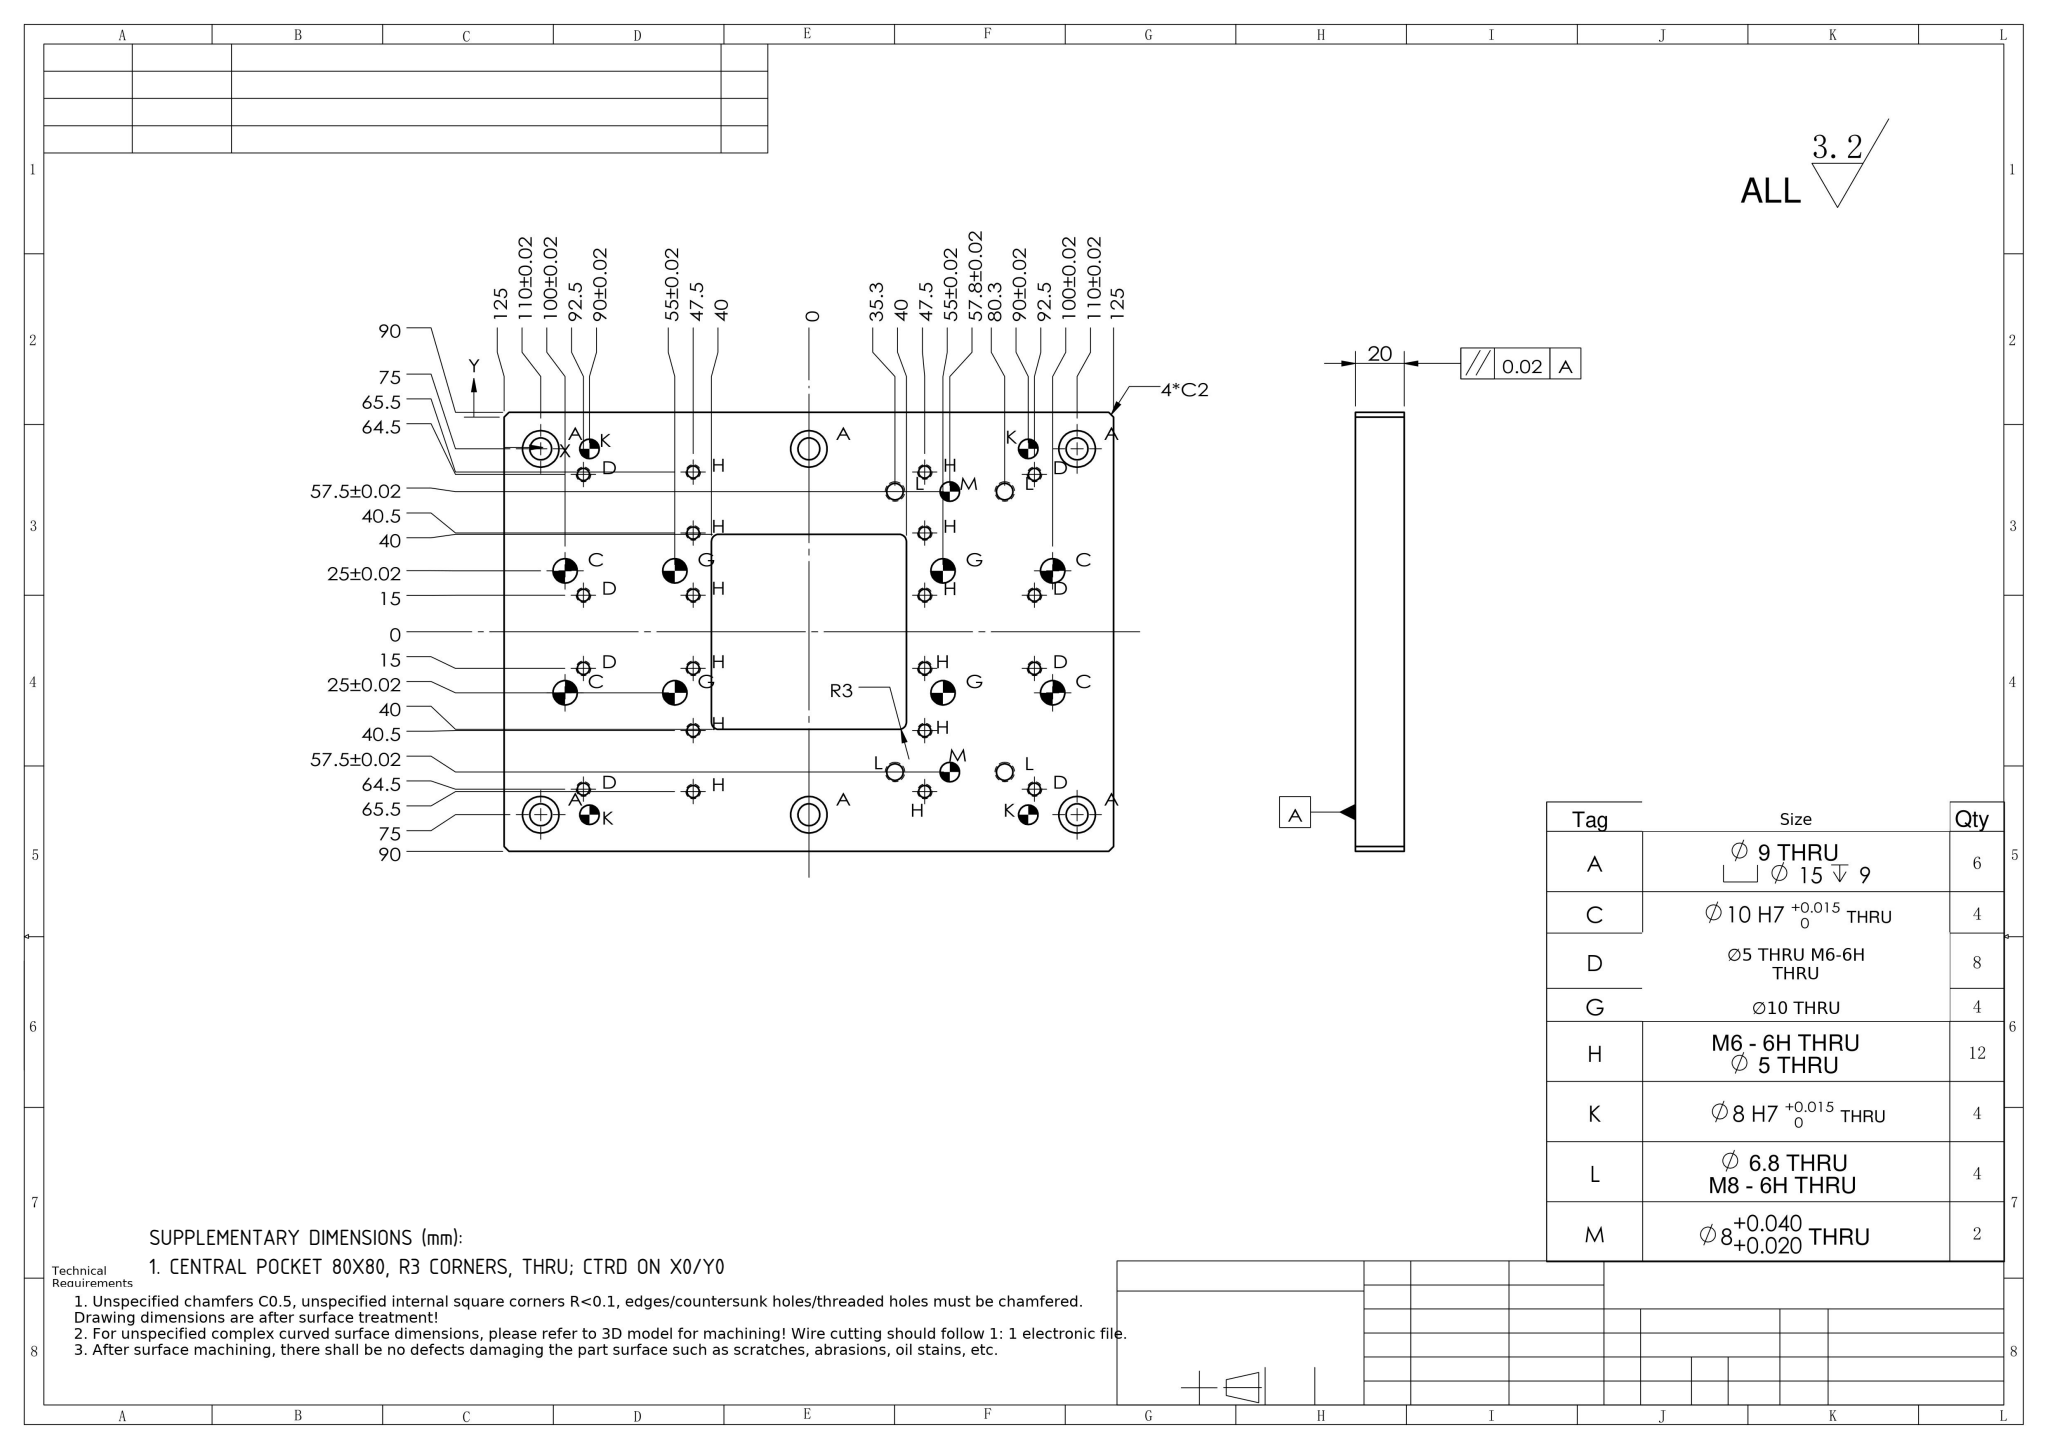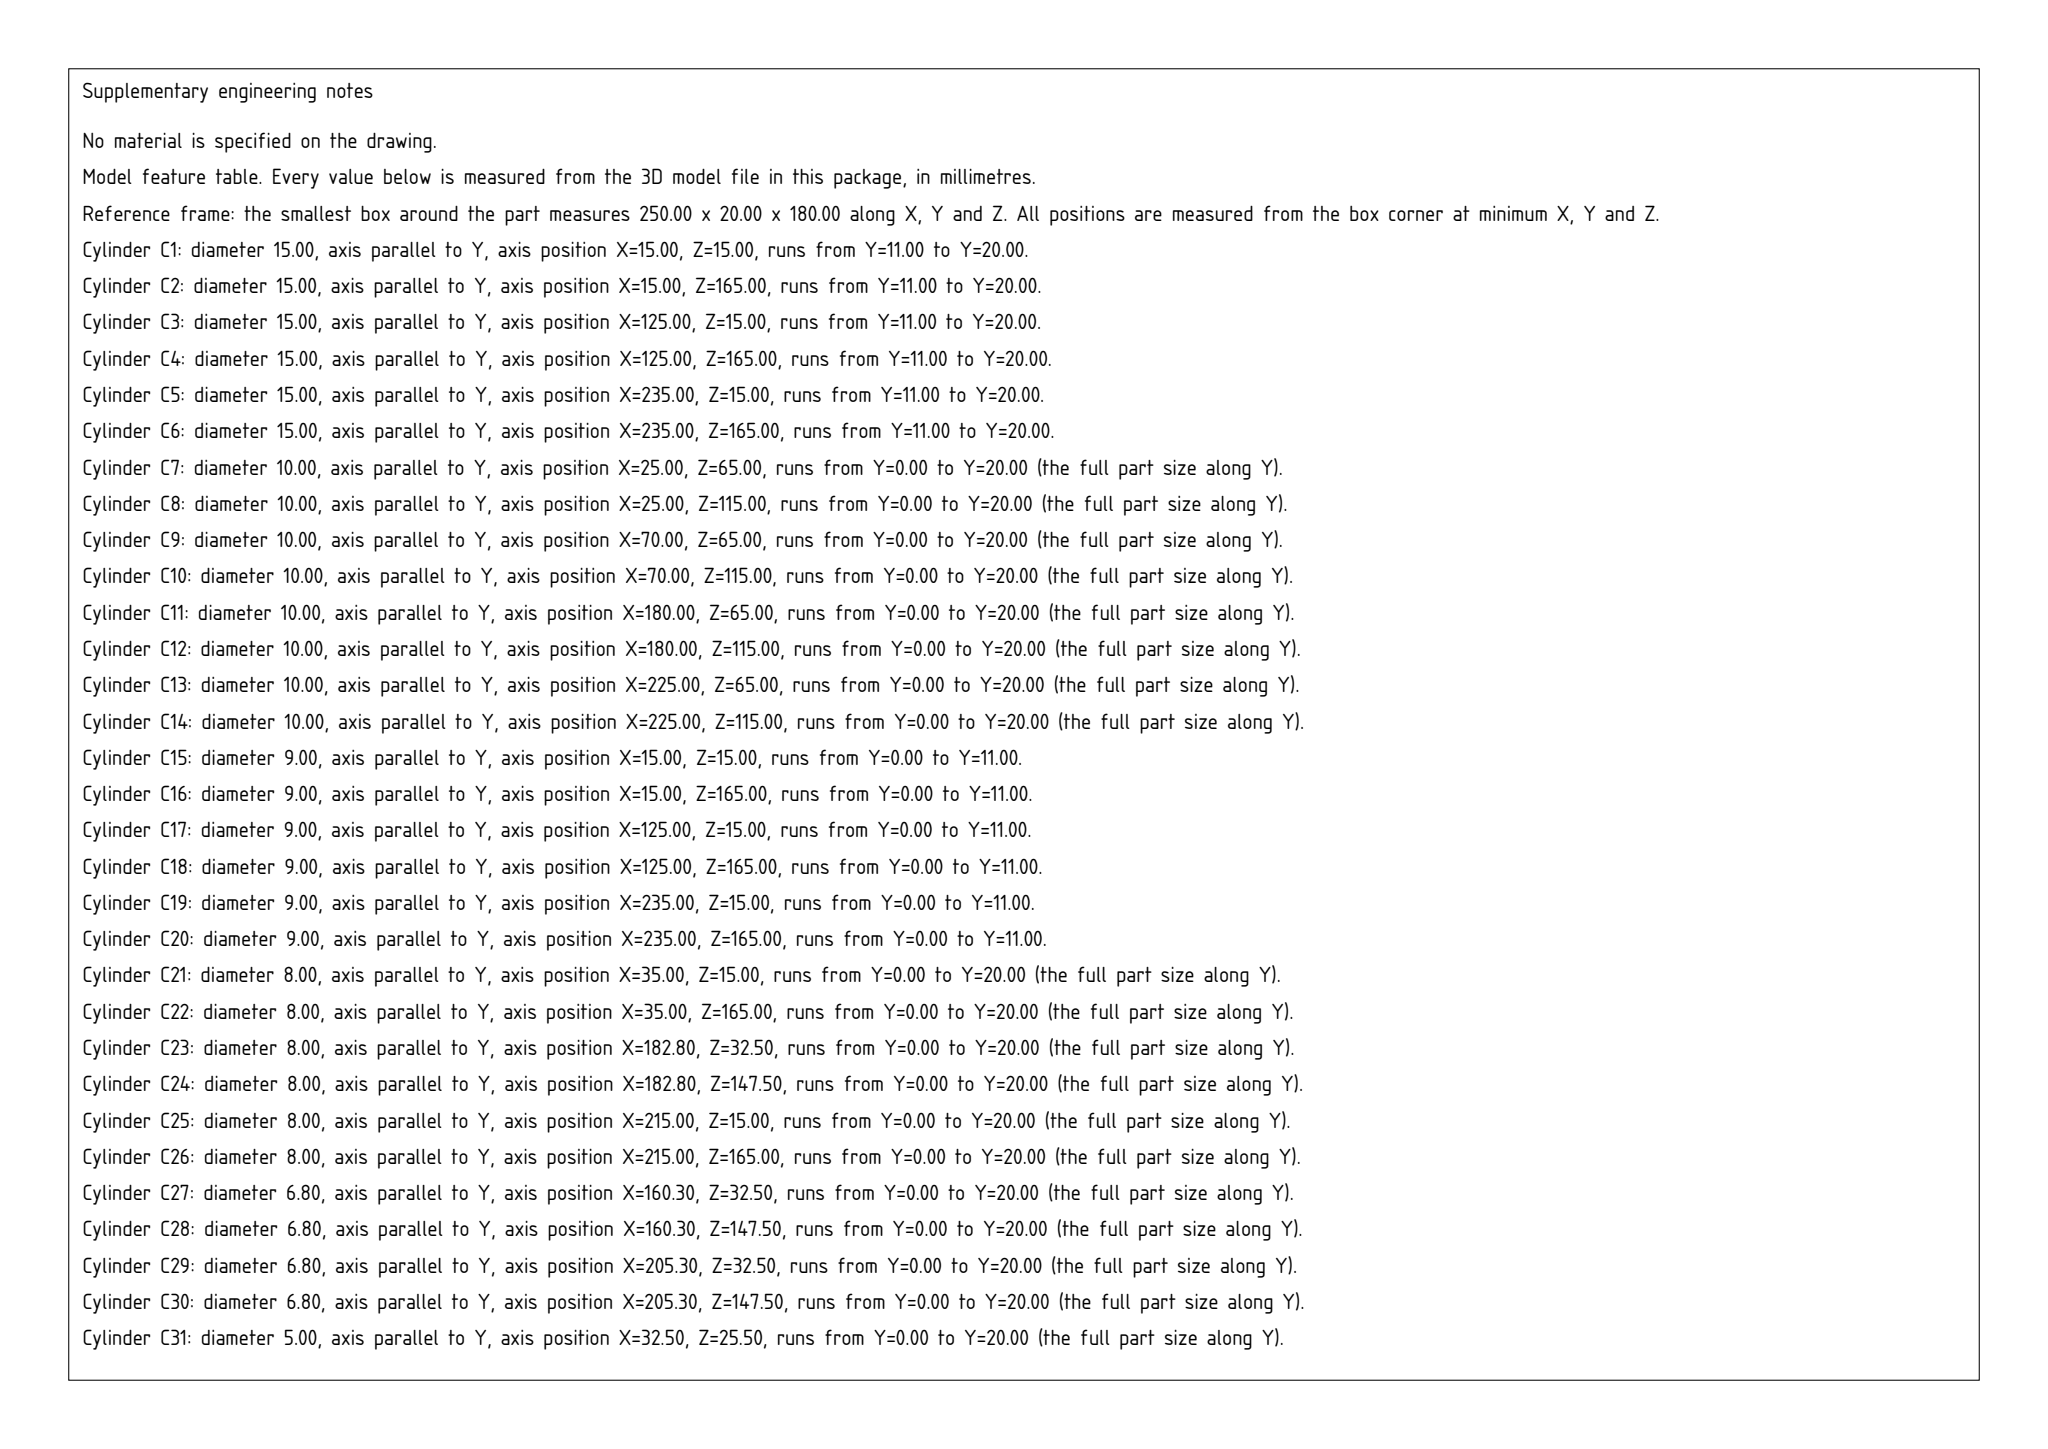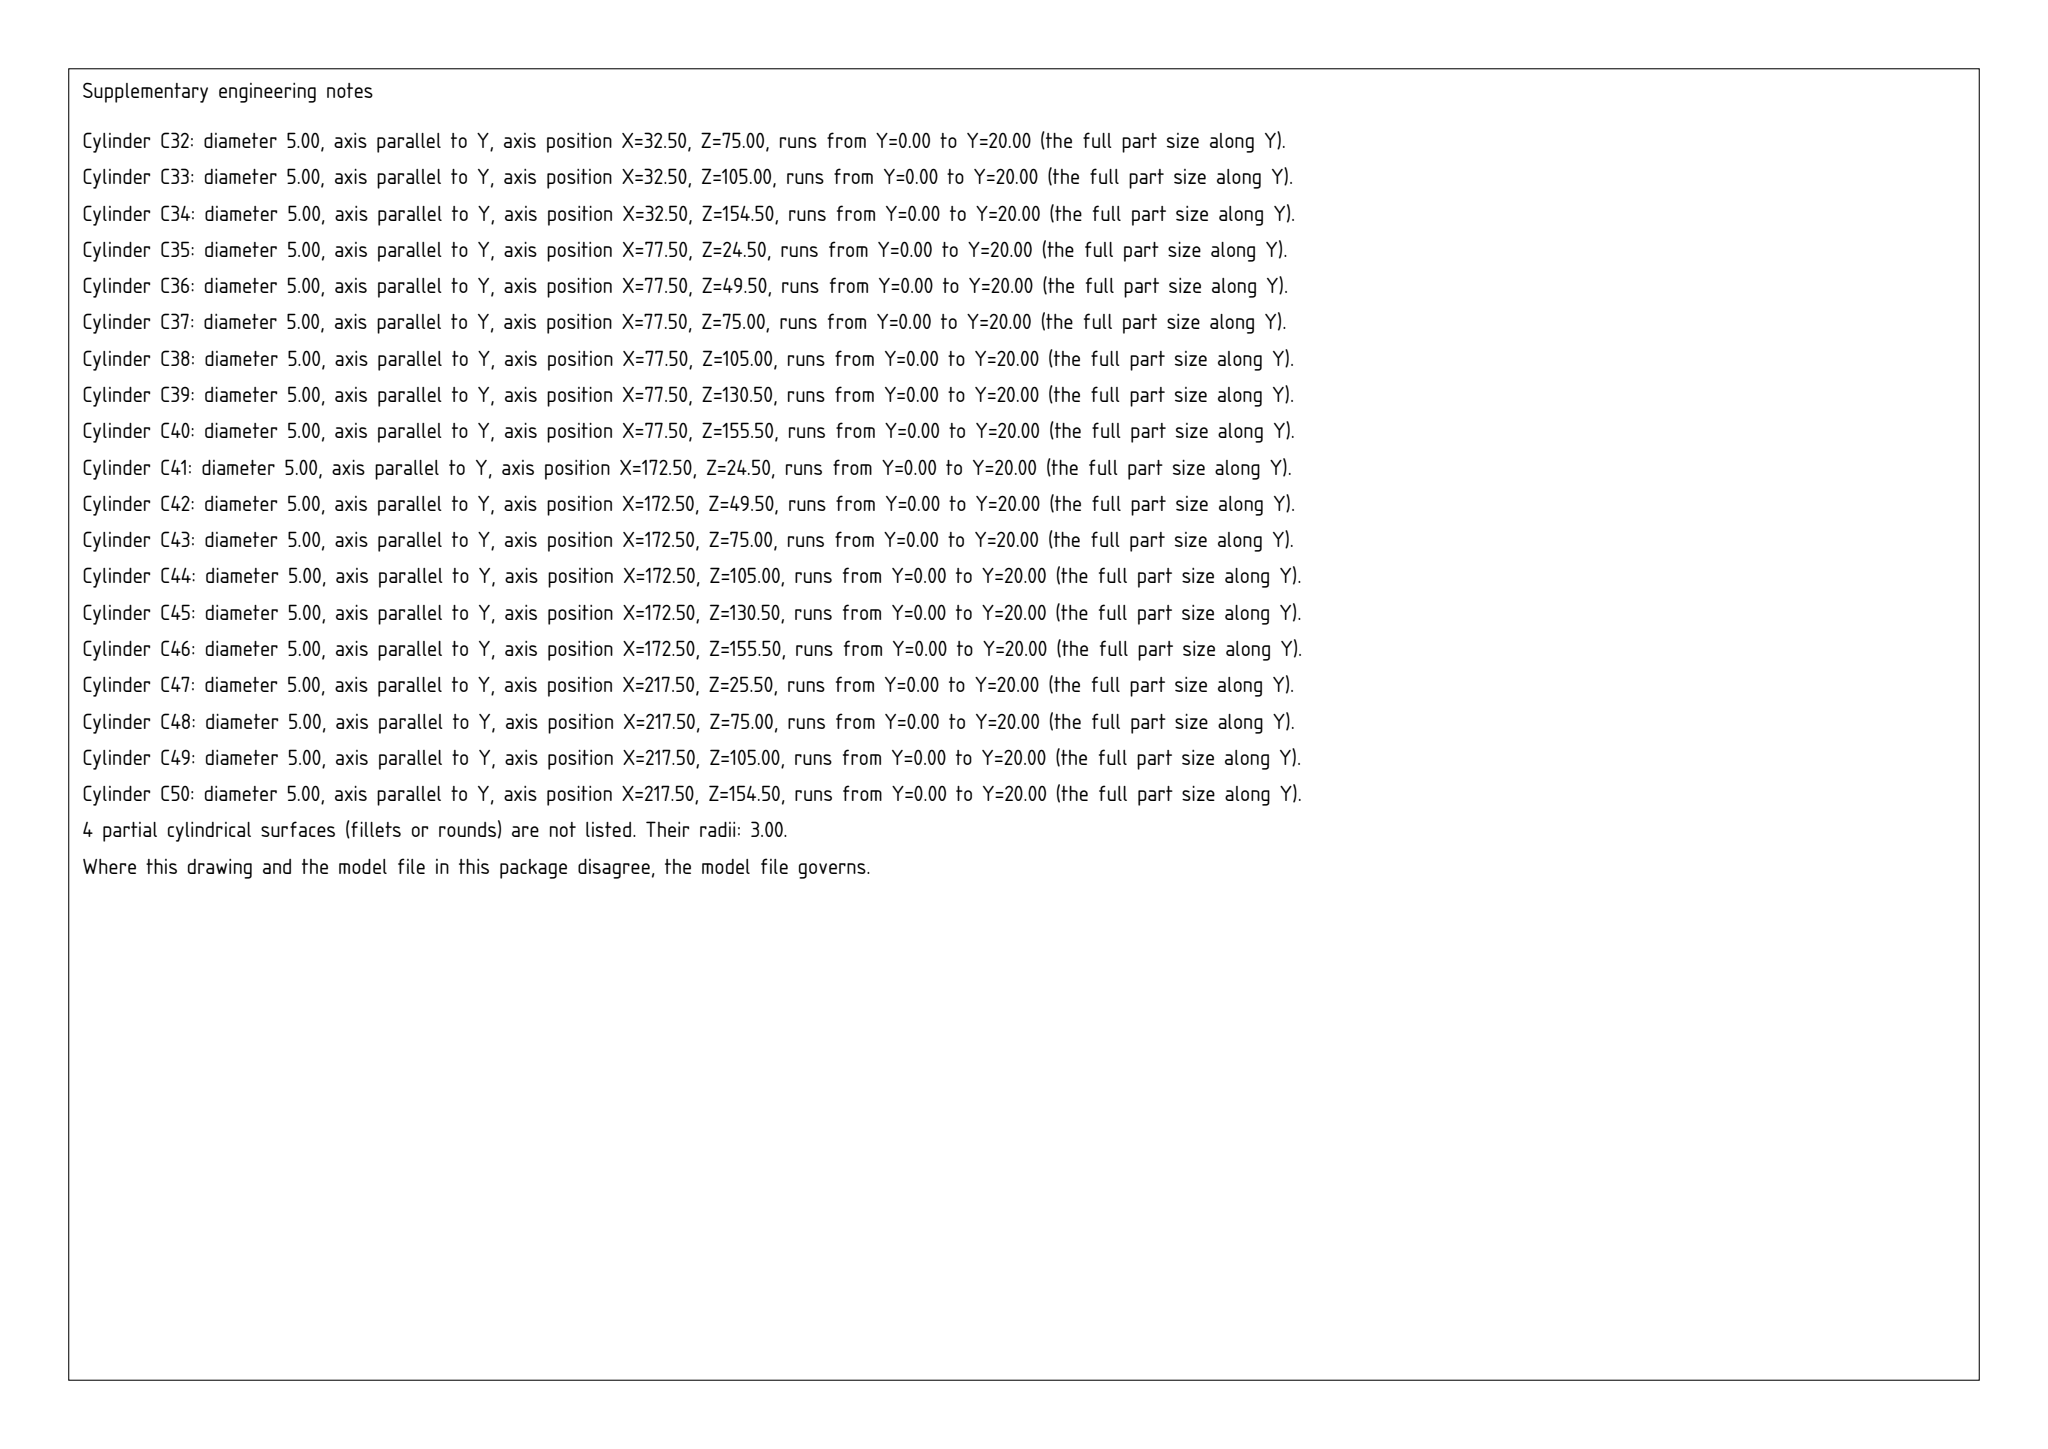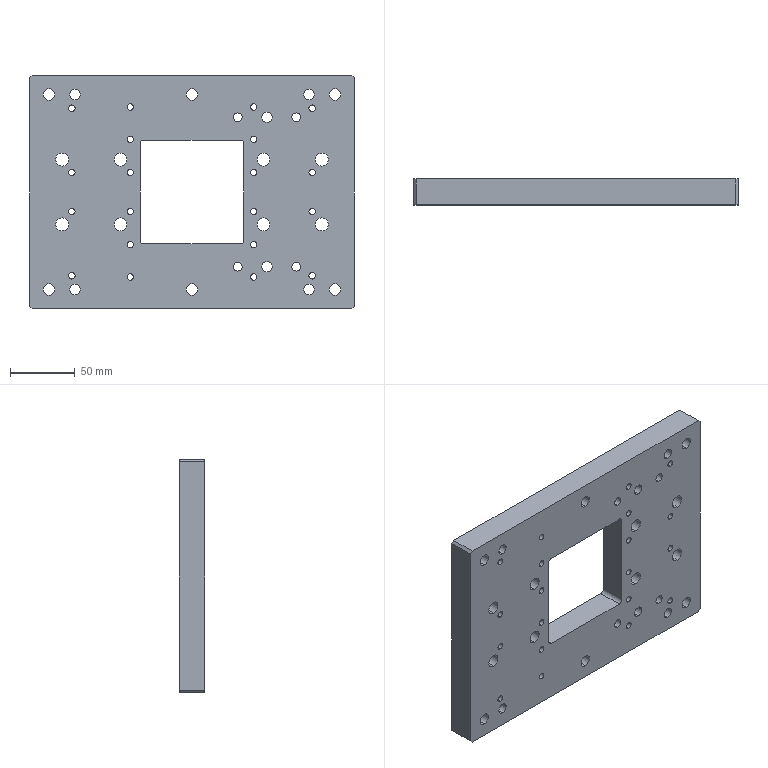Part | SolidWorks | mm | 1 solid | 124 faces | box 250 x 20 x 180 mm | volume 728896 mm3 | cylinder 104 | plane 20 | commonest cylinder face diameters 5 x40 10 x16 8 x12 15 x12 9 x12 6.8 x8 6 x4
build123d program:
from build123d import *

# Parameters (mm, degrees)
SKETCH1_W                                           = 250
SKETCH1_H                                           = 180
SKETCH1_W_2                                         = 80
SKETCH1_H_2                                         = 80
BOSS_EXTRUDE1_DEPTH                                 = 20
FILLET1_R                                           = 3
CHAMFER2_SIZE                                       = 2
SKETCH3_R                                           = 5
CUT_EXTRUDE1_DEPTH                                  = 45
M6_TAPPED_HOLE1_D                                   = 5
SIZE_MM_DOWEL_PIN_HOLE0_D                           = 8
M8_TAPPED_HOLE1_D                                   = 6.8
HOLE_SIZE_ACCORDING_TO_TYPE1_OF_HEXAGON_D           = 9
HOLE_SIZE_ACCORDING_TO_TYPE1_OF_HEXAGON_CBORE_D     = 15
HOLE_SIZE_ACCORDING_TO_TYPE1_OF_HEXAGON_CBORE_DEPTH = 9
SIZE_MM_CLEARANCE_DOWEL_PIN_HOLE1_D                 = 10
M6_TAPPED_HOLE2_D                                   = 5
M6_TAPPED_HOLE3_D                                   = 5
SKETCH10_R                                          = 4
CUT_EXTRUDE2_DEPTH                                  = 156.322


with BuildPart() as part:
    # Sketch1 → Boss-Extrude1 (new body)
    with BuildSketch(Plane(origin=(0, 0, 0), x_dir=(1, 0, 0), z_dir=(0, 1, 0))):
        Rectangle(SKETCH1_W, SKETCH1_H)
        Rectangle(SKETCH1_W_2, SKETCH1_H_2, mode=Mode.SUBTRACT)
    extrude(amount=BOSS_EXTRUDE1_DEPTH)

    # Fillet1
    fillet1_edges = [part.edges().sort_by_distance(p)[0] for p in [
        (40, 10, 40),
        (40, 10, -40),
        (-40, 10, -40),
        (-40, 10, 40),
    ]]
    fillet(fillet1_edges, radius=FILLET1_R)

    # Chamfer2
    chamfer2_edges = [part.edges().sort_by_distance(p)[0] for p in [
        (125, 10, 90),
        (-125, 10, 90),
        (-125, 10, -90),
        (125, 10, -90),
    ]]
    chamfer(chamfer2_edges, length=CHAMFER2_SIZE)

    # Sketch3 → Cut-Extrude1 (cut)
    with BuildSketch(Plane(origin=(0, 20, 0), x_dir=(1, 0, 0), z_dir=(0, 1, 0))):
        with Locations(Location((-100, 25, 0), (0, 0, 270))):
            Circle(SKETCH3_R)
        with Locations(Location((-100, -25, 0), (0, 0, 270))):
            Circle(SKETCH3_R)
        with Locations(Location((100, 25, 0), (0, 0, 270))):
            Circle(SKETCH3_R)
        with Locations(Location((100, -25, 0), (0, 0, 270))):
            Circle(SKETCH3_R)
    extrude(amount=-CUT_EXTRUDE1_DEPTH, mode=Mode.SUBTRACT)

    # M6 Tapped Hole1 (through all)
    with Locations(Plane(origin=(0, 20, 0), x_dir=(1, 0, 0), z_dir=(0, 1, 0))):
        with Locations((92.5, 64.5), (92.5, -64.5), (-92.5, -64.5), (-92.5, 64.5), (-92.5, 15), (-92.5, -15), (92.5, 15), (92.5, -15)):
            Hole(M6_TAPPED_HOLE1_D / 2)

    # Size mm Dowel Pin Hole0 (through all)
    with Locations(Plane(origin=(0, 0, 0), x_dir=(-1, 0, 0), z_dir=(0, -1, 0))):
        with Locations((-57.8, 57.5), (-57.8, -57.5)):
            Hole(SIZE_MM_DOWEL_PIN_HOLE0_D / 2)

    # M8 Tapped Hole1 (through all)
    with Locations(Plane(origin=(0, 0, 0), x_dir=(-1, 0, 0), z_dir=(0, -1, 0))):
        with Locations((-35.3, 57.5), (-80.3, 57.5), (-35.3, -57.5), (-80.3, -57.5)):
            Hole(M8_TAPPED_HOLE1_D / 2)

    # Hole Size_ according to_Type1 of Hexagon (through all)
    with Locations(Plane(origin=(0, 20, 0), x_dir=(1, 0, 0), z_dir=(0, 1, 0))):
        with Locations((-110, 75), (110, 75), (110, -75), (-110, -75), (0, 75), (0, -75)):
            CounterBoreHole(HOLE_SIZE_ACCORDING_TO_TYPE1_OF_HEXAGON_D / 2, HOLE_SIZE_ACCORDING_TO_TYPE1_OF_HEXAGON_CBORE_D / 2, HOLE_SIZE_ACCORDING_TO_TYPE1_OF_HEXAGON_CBORE_DEPTH)

    # Size mm Clearance Dowel Pin Hole1 (through all)
    with Locations(Plane(origin=(0, 20, 0), x_dir=(1, 0, 0), z_dir=(0, 1, 0))):
        with Locations((55, -25), (55, 25), (-55, -25), (-55, 25)):
            Hole(SIZE_MM_CLEARANCE_DOWEL_PIN_HOLE1_D / 2)

    # M6 Tapped Hole2 (through all)
    with Locations(Plane(origin=(0, 20, 0), x_dir=(1, 0, 0), z_dir=(0, 1, 0))):
        with Locations((47.5, -40.5), (47.5, -15), (47.5, 15), (47.5, 40.5), (-47.5, 40.5), (-47.5, -40.5), (-47.5, -15), (-47.5, 15)):
            Hole(M6_TAPPED_HOLE2_D / 2)

    # M6 Tapped Hole3 (through all)
    with Locations(Plane(origin=(0, 20, 0), x_dir=(1, 0, 0), z_dir=(0, 1, 0))):
        with Locations((47.5, -65.5), (-47.5, -65.5), (47.5, 65.5), (-47.5, 65.5)):
            Hole(M6_TAPPED_HOLE3_D / 2)

    # Sketch10 → Cut-Extrude2 (cut, through all)
    with BuildSketch(Plane(origin=(0, 20, 0), x_dir=(1, 0, 0), z_dir=(0, 1, 0))):
        with Locations(Location((-90, 75, 0), (0, 0, 270))):
            Circle(SKETCH10_R)
        with Locations(Location((90, 75, 0), (0, 0, 270))):
            Circle(SKETCH10_R)
        with Locations(Location((90, -75, 0), (0, 0, 90))):
            Circle(SKETCH10_R)
        with Locations(Location((-90, -75, 0), (0, 0, 90))):
            Circle(SKETCH10_R)
    extrude(amount=-CUT_EXTRUDE2_DEPTH, mode=Mode.SUBTRACT)


solid = part.part